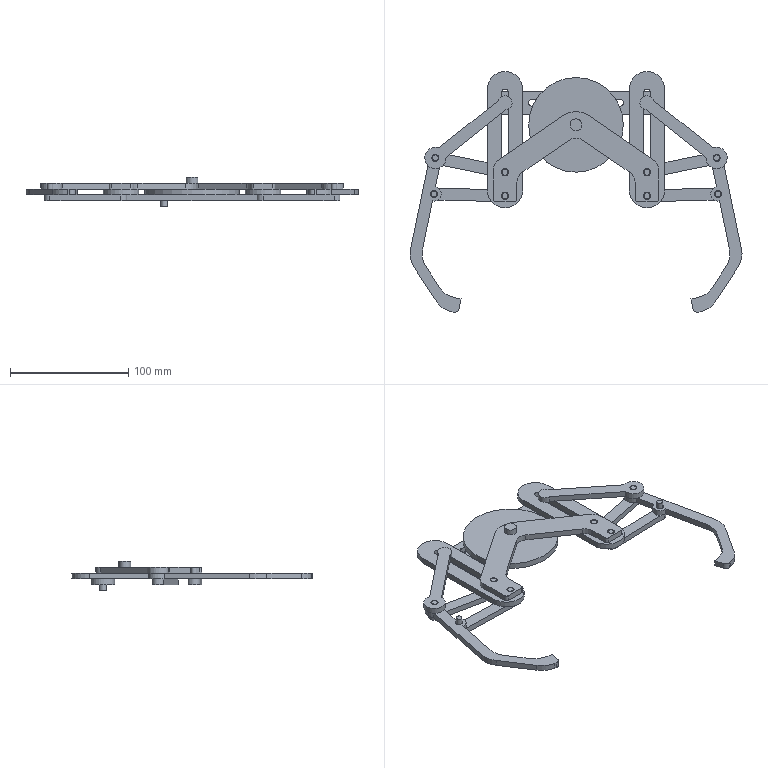Assembly | NX | mm | 13 component files | 13 solids | 166 faces | box 280.54 x 203.37 x 25 mm | volume 125147 mm3 | plane 88 | cylinder 78 | commonest cylinder face diameters 6 x25 10 x10 40 x9 5 x8 20 x7 12 x4 4 x4 30 x4
Bill of materials:
unnamed part 1 | 1 |  | Thin circular disc with a short cylindrical pin rising from the center of one face and a smaller cylindrical pin projecting from the opposite face at an off-center position.
unnamed part 2 | 4 |  | Straight flat bar with fully rounded (obround) ends and a cylindrical pin standing up from the same face near each end.
unnamed part 3 | 2 |  | Slender flat link with a round eye containing a through-hole at one end and a rounded end at the other end carrying a cylindrical pin that projects from one face.
unnamed part 4 | 2 |  | Flat obround plate with a long straight slot along its centerline and two round through-holes lined up with the slot near one end.
unnamed part 5 | 2 |  | Flat, curved lever-like arm with a straight section ending in a round boss with a through-hole, a second side boss with a hole partway along, and a curved hooked tail ending in a blunt cut end.
unnamed part 6 | 1 |  | Flat plate shaped like an inverted V (chevron) with two parallel straight legs, a large through-hole at the rounded apex, and two small through-holes in each leg end.
unnamed part 7 | 1 |  | Flat obround strap with a long central through-slot and one small round through-hole near each rounded end.
Mates:
1. fix | lower_conn_plate 1 component
2. center | ball_head_waist_plate 2 face | ball_head_waist_plate 2 face | lower_conn_plate 1 face
3. touch align | lower_conn_plate 1 face | ball_head_waist_plate 2 face
4. touch align | ball_head_waist_plate 1 face | lower_conn_plate 1 face
5. center | ball_head_waist_plate 1 face | ball_head_waist_plate 1 face | lower_conn_plate 1 face
6. touch align | round_disc 1 face | lower_conn_plate 1 face
7. center | lower_conn_plate 1 face | lower_conn_plate 1 face | round_disc 1 face
8. concentric | upper_conn_plate 1 edge | round_disc 1 edge
9. concentric | upper_conn_plate 1 edge | ball_head_waist_plate 2 edge
10. concentric | upper_conn_plate 1 edge | ball_head_waist_plate 1 edge
11. concentric | upper_conn_plate 1 edge | ball_head_waist_plate 2 edge
12. concentric | upper_conn_plate 1 edge | ball_head_waist_plate 1 edge
13. concentric | conn_rod 4 arc | ball_head_waist_plate 2 edge
14. concentric | conn_rod 3 arc | ball_head_waist_plate 2 edge
15. concentric | conn_rod 2 arc | ball_head_waist_plate 1 edge
16. concentric | conn_rod 1 arc | ball_head_waist_plate 1 edge
17. touch align | conn_arm 2 face | lower_conn_plate 1 face
18. concentric | conn_arm 2 arc | conn_rod 4 edge
19. touch align | conn_arm 1 face | lower_conn_plate 1 face
20. concentric | conn_arm 1 arc | conn_rod 2 edge
21. concentric | clamp_arm 2 arc | conn_rod 4 edge
22. touch align | clamp_arm 2 face | conn_rod 3 face
23. concentric | clamp_arm 1 edge | conn_rod 2 edge
24. touch align | clamp_arm 1 face | conn_rod 1 face